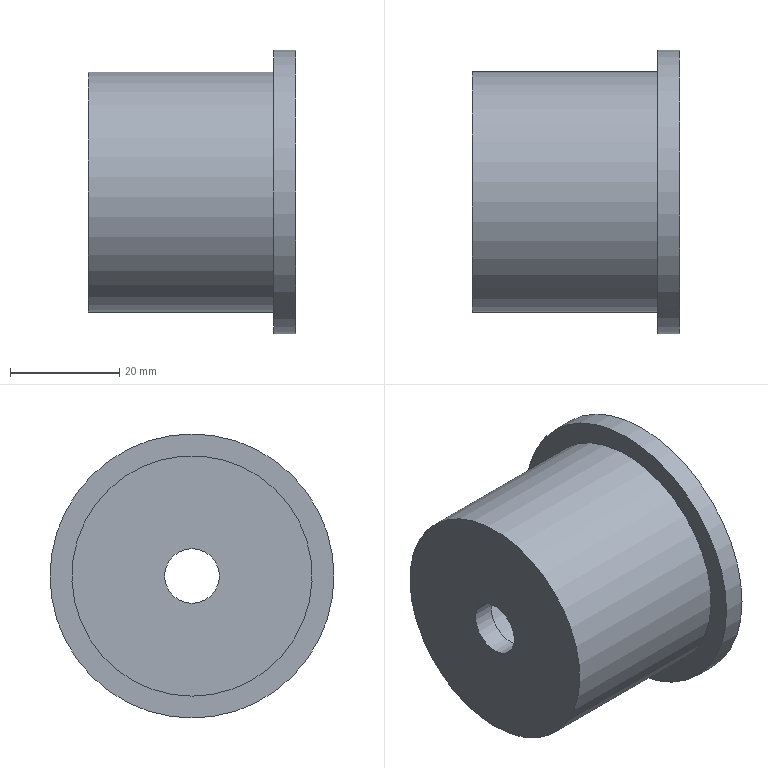Component | NX | LARGE_SPRING_BASE_2 | 1 solid | 10 faces | box 38 x 52 x 52 mm | volume 38909 mm3 | plane 5 | cylinder 5 | commonest cylinder face diameters 10 x1 26 x1 36 x1 52 x1 44 x1
STEP:
#1=CARTESIAN_POINT('',(0.,0.,0.));
#2=DIRECTION('',(0.,0.,1.));
#3=DIRECTION('',(1.,0.,0.));
#4=AXIS2_PLACEMENT_3D('',#1,#2,#3);
#5=CARTESIAN_POINT('',(-43.003,0.,-5.));
#6=VERTEX_POINT('',#5);
#7=CARTESIAN_POINT('',(-43.003,0.,0.));
#8=DIRECTION('',(-1.,0.,0.));
#9=DIRECTION('',(0.,0.,-1.));
#10=AXIS2_PLACEMENT_3D('',#7,#8,#9);
#11=CIRCLE('',#10,5.);
#12=CARTESIAN_POINT('',(-43.003,0.,22.));
#13=DIRECTION('',(1.,0.,0.));
#14=DIRECTION('',(0.,0.,1.));
#15=AXIS2_PLACEMENT_3D('',#12,#13,#14);
#16=PLANE('',#15);
#17=CARTESIAN_POINT('',(-27.,0.));
#18=CARTESIAN_POINT('',(-27.,8.66));
#19=CARTESIAN_POINT('',(-19.5,4.33));
#20=CARTESIAN_POINT('',(-12.,0.));
#21=CARTESIAN_POINT('',(-19.5,-4.33));
#22=CARTESIAN_POINT('',(-27.,-8.66));
#23=CARTESIAN_POINT('',(-27.,0.));
#24=(BOUNDED_CURVE()B_SPLINE_CURVE(2,(#17,#18,#19,#20,#21,#22,#23),.UNSPECIFIED.,.T.,.F.)B_SPLINE_CURVE_WITH_KNOTS((1,2,2,2,2,1),(-2.094,0.,2.094,4.189,6.283,8.378),.UNSPECIFIED.)CURVE()GEOMETRIC_REPRESENTATION_ITEM()RATIONAL_B_SPLINE_CURVE((1.,0.5,1.,0.5,1.,0.5,1.))REPRESENTATION_ITEM(''));
#25=(GEOMETRIC_REPRESENTATION_CONTEXT(2)PARAMETRIC_REPRESENTATION_CONTEXT()REPRESENTATION_CONTEXT('',''));
#26=DEFINITIONAL_REPRESENTATION('',(#24),#25);
#27=PCURVE('',#16,#26);
#28=CARTESIAN_POINT('',(-5.,0.,0.));
#29=DIRECTION('',(-1.,0.,0.));
#30=DIRECTION('',(0.,0.,-1.));
#31=AXIS2_PLACEMENT_3D('',#28,#29,#30);
#32=CYLINDRICAL_SURFACE('',#31,5.);
#33=CARTESIAN_POINT('',(0.,38.003));
#34=DIRECTION('',(1.,0.));
#35=VECTOR('',#34,1.);
#36=LINE('',#33,#35);
#37=(GEOMETRIC_REPRESENTATION_CONTEXT(2)PARAMETRIC_REPRESENTATION_CONTEXT()REPRESENTATION_CONTEXT('',''));
#38=DEFINITIONAL_REPRESENTATION('',(#36),#37);
#39=PCURVE('',#32,#38);
#40=SURFACE_CURVE('',#11,(#27,#39),.PCURVE_S1.);
#41=EDGE_CURVE('',#6,#6,#40,.T.);
#42=ORIENTED_EDGE('',*,*,#41,.F.);
#43=EDGE_LOOP('',(#42));
#44=FACE_BOUND('',#43,.T.);
#45=CARTESIAN_POINT('',(-43.003,0.,-22.));
#46=VERTEX_POINT('',#45);
#47=CARTESIAN_POINT('',(-43.003,0.,0.));
#48=DIRECTION('',(-1.,0.,0.));
#49=DIRECTION('',(0.,0.,-1.));
#50=AXIS2_PLACEMENT_3D('',#47,#48,#49);
#51=CIRCLE('',#50,22.);
#52=CARTESIAN_POINT('',(-44.,0.));
#53=CARTESIAN_POINT('',(-44.,38.105));
#54=CARTESIAN_POINT('',(-11.,19.053));
#55=CARTESIAN_POINT('',(22.,0.));
#56=CARTESIAN_POINT('',(-11.,-19.053));
#57=CARTESIAN_POINT('',(-44.,-38.105));
#58=CARTESIAN_POINT('',(-44.,0.));
#59=(BOUNDED_CURVE()B_SPLINE_CURVE(2,(#52,#53,#54,#55,#56,#57,#58),.UNSPECIFIED.,.T.,.F.)B_SPLINE_CURVE_WITH_KNOTS((1,2,2,2,2,1),(-2.094,0.,2.094,4.189,6.283,8.378),.UNSPECIFIED.)CURVE()GEOMETRIC_REPRESENTATION_ITEM()RATIONAL_B_SPLINE_CURVE((1.,0.5,1.,0.5,1.,0.5,1.))REPRESENTATION_ITEM(''));
#60=(GEOMETRIC_REPRESENTATION_CONTEXT(2)PARAMETRIC_REPRESENTATION_CONTEXT()REPRESENTATION_CONTEXT('',''));
#61=DEFINITIONAL_REPRESENTATION('',(#59),#60);
#62=PCURVE('',#16,#61);
#63=CARTESIAN_POINT('',(-5.,0.,0.));
#64=DIRECTION('',(-1.,0.,0.));
#65=DIRECTION('',(0.,0.,-1.));
#66=AXIS2_PLACEMENT_3D('',#63,#64,#65);
#67=CYLINDRICAL_SURFACE('',#66,22.);
#68=CARTESIAN_POINT('',(0.,38.003));
#69=DIRECTION('',(1.,0.));
#70=VECTOR('',#69,1.);
#71=LINE('',#68,#70);
#72=(GEOMETRIC_REPRESENTATION_CONTEXT(2)PARAMETRIC_REPRESENTATION_CONTEXT()REPRESENTATION_CONTEXT('',''));
#73=DEFINITIONAL_REPRESENTATION('',(#71),#72);
#74=PCURVE('',#67,#73);
#75=SURFACE_CURVE('',#51,(#62,#74),.PCURVE_S1.);
#76=EDGE_CURVE('',#46,#46,#75,.T.);
#77=ORIENTED_EDGE('',*,*,#76,.T.);
#78=EDGE_LOOP('',(#77));
#79=FACE_BOUND('',#78,.T.);
#80=ADVANCED_FACE('',(#44,#79),#16,.F.);
#81=CARTESIAN_POINT('',(-39.003,0.,-5.));
#82=VERTEX_POINT('',#81);
#83=CARTESIAN_POINT('',(-39.003,0.,0.));
#84=DIRECTION('',(-1.,0.,0.));
#85=DIRECTION('',(0.,0.,-1.));
#86=AXIS2_PLACEMENT_3D('',#83,#84,#85);
#87=CIRCLE('',#86,5.);
#88=CARTESIAN_POINT('',(0.,34.003));
#89=DIRECTION('',(1.,0.));
#90=VECTOR('',#89,1.);
#91=LINE('',#88,#90);
#92=(GEOMETRIC_REPRESENTATION_CONTEXT(2)PARAMETRIC_REPRESENTATION_CONTEXT()REPRESENTATION_CONTEXT('',''));
#93=DEFINITIONAL_REPRESENTATION('',(#91),#92);
#94=PCURVE('',#32,#93);
#95=CARTESIAN_POINT('',(-39.003,0.,5.));
#96=DIRECTION('',(-1.,0.,0.));
#97=DIRECTION('',(0.,0.,-1.));
#98=AXIS2_PLACEMENT_3D('',#95,#96,#97);
#99=PLANE('',#98);
#100=CARTESIAN_POINT('',(5.,0.));
#101=DIRECTION('',(1.,0.));
#102=AXIS2_PLACEMENT_2D('',#100,#101);
#103=CIRCLE('',#102,5.);
#104=(GEOMETRIC_REPRESENTATION_CONTEXT(2)PARAMETRIC_REPRESENTATION_CONTEXT()REPRESENTATION_CONTEXT('',''));
#105=DEFINITIONAL_REPRESENTATION('',(#103),#104);
#106=PCURVE('',#99,#105);
#107=SURFACE_CURVE('',#87,(#94,#106),.PCURVE_S1.);
#108=EDGE_CURVE('',#82,#82,#107,.T.);
#109=ORIENTED_EDGE('',*,*,#108,.T.);
#110=CARTESIAN_POINT('',(-39.003,0.,-5.));
#111=CARTESIAN_POINT('',(-43.003,0.,-5.));
#112=B_SPLINE_CURVE_WITH_KNOTS('',1,(#110,#111),.UNSPECIFIED.,.F.,.F.,(2,2),(34.003,38.003),.PIECEWISE_BEZIER_KNOTS.);
#113=CARTESIAN_POINT('',(6.283,0.));
#114=DIRECTION('',(0.,1.));
#115=VECTOR('',#114,1.);
#116=LINE('',#113,#115);
#117=(GEOMETRIC_REPRESENTATION_CONTEXT(2)PARAMETRIC_REPRESENTATION_CONTEXT()REPRESENTATION_CONTEXT('',''));
#118=DEFINITIONAL_REPRESENTATION('',(#116),#117);
#119=PCURVE('',#32,#118);
#120=CARTESIAN_POINT('',(0.,0.));
#121=DIRECTION('',(0.,1.));
#122=VECTOR('',#121,1.);
#123=LINE('',#120,#122);
#124=(GEOMETRIC_REPRESENTATION_CONTEXT(2)PARAMETRIC_REPRESENTATION_CONTEXT()REPRESENTATION_CONTEXT('',''));
#125=DEFINITIONAL_REPRESENTATION('',(#123),#124);
#126=PCURVE('',#32,#125);
#127=SEAM_CURVE('',#112,(#119,#126),.PCURVE_S1.);
#128=EDGE_CURVE('',#82,#6,#127,.T.);
#129=ORIENTED_EDGE('',*,*,#128,.T.);
#130=ORIENTED_EDGE('',*,*,#41,.F.);
#131=ORIENTED_EDGE('',*,*,#128,.F.);
#132=EDGE_LOOP('',(#109,#129,#130,#131));
#133=FACE_BOUND('',#132,.F.);
#134=ADVANCED_FACE('',(#133),#32,.F.);
#135=CARTESIAN_POINT('',(-39.003,0.,-13.));
#136=VERTEX_POINT('',#135);
#137=CARTESIAN_POINT('',(-39.003,0.,0.));
#138=DIRECTION('',(-1.,0.,0.));
#139=DIRECTION('',(0.,0.,-1.));
#140=AXIS2_PLACEMENT_3D('',#137,#138,#139);
#141=CIRCLE('',#140,13.);
#142=CARTESIAN_POINT('',(5.,0.));
#143=DIRECTION('',(1.,0.));
#144=AXIS2_PLACEMENT_2D('',#142,#143);
#145=CIRCLE('',#144,13.);
#146=(GEOMETRIC_REPRESENTATION_CONTEXT(2)PARAMETRIC_REPRESENTATION_CONTEXT()REPRESENTATION_CONTEXT('',''));
#147=DEFINITIONAL_REPRESENTATION('',(#145),#146);
#148=PCURVE('',#99,#147);
#149=CARTESIAN_POINT('',(-5.,0.,0.));
#150=DIRECTION('',(-1.,0.,0.));
#151=DIRECTION('',(0.,0.,-1.));
#152=AXIS2_PLACEMENT_3D('',#149,#150,#151);
#153=CYLINDRICAL_SURFACE('',#152,13.);
#154=CARTESIAN_POINT('',(0.,34.003));
#155=DIRECTION('',(1.,0.));
#156=VECTOR('',#155,1.);
#157=LINE('',#154,#156);
#158=(GEOMETRIC_REPRESENTATION_CONTEXT(2)PARAMETRIC_REPRESENTATION_CONTEXT()REPRESENTATION_CONTEXT('',''));
#159=DEFINITIONAL_REPRESENTATION('',(#157),#158);
#160=PCURVE('',#153,#159);
#161=SURFACE_CURVE('',#141,(#148,#160),.PCURVE_S1.);
#162=EDGE_CURVE('',#136,#136,#161,.T.);
#163=ORIENTED_EDGE('',*,*,#162,.F.);
#164=EDGE_LOOP('',(#163));
#165=FACE_BOUND('',#164,.T.);
#166=ORIENTED_EDGE('',*,*,#108,.T.);
#167=EDGE_LOOP('',(#166));
#168=FACE_BOUND('',#167,.T.);
#169=ADVANCED_FACE('',(#165,#168),#99,.F.);
#170=CARTESIAN_POINT('',(-11.003,0.,-13.));
#171=VERTEX_POINT('',#170);
#172=CARTESIAN_POINT('',(-11.003,0.,0.));
#173=DIRECTION('',(-1.,0.,0.));
#174=DIRECTION('',(0.,0.,-1.));
#175=AXIS2_PLACEMENT_3D('',#172,#173,#174);
#176=CIRCLE('',#175,13.);
#177=CARTESIAN_POINT('',(0.,6.003));
#178=DIRECTION('',(1.,0.));
#179=VECTOR('',#178,1.);
#180=LINE('',#177,#179);
#181=(GEOMETRIC_REPRESENTATION_CONTEXT(2)PARAMETRIC_REPRESENTATION_CONTEXT()REPRESENTATION_CONTEXT('',''));
#182=DEFINITIONAL_REPRESENTATION('',(#180),#181);
#183=PCURVE('',#153,#182);
#184=CARTESIAN_POINT('',(-11.003,0.,13.));
#185=DIRECTION('',(-1.,0.,0.));
#186=DIRECTION('',(0.,0.,-1.));
#187=AXIS2_PLACEMENT_3D('',#184,#185,#186);
#188=PLANE('',#187);
#189=CARTESIAN_POINT('',(13.,0.));
#190=DIRECTION('',(1.,0.));
#191=AXIS2_PLACEMENT_2D('',#189,#190);
#192=CIRCLE('',#191,13.);
#193=(GEOMETRIC_REPRESENTATION_CONTEXT(2)PARAMETRIC_REPRESENTATION_CONTEXT()REPRESENTATION_CONTEXT('',''));
#194=DEFINITIONAL_REPRESENTATION('',(#192),#193);
#195=PCURVE('',#188,#194);
#196=SURFACE_CURVE('',#176,(#183,#195),.PCURVE_S1.);
#197=EDGE_CURVE('',#171,#171,#196,.T.);
#198=ORIENTED_EDGE('',*,*,#197,.T.);
#199=CARTESIAN_POINT('',(-11.003,0.,-13.));
#200=CARTESIAN_POINT('',(-39.003,0.,-13.));
#201=B_SPLINE_CURVE_WITH_KNOTS('',1,(#199,#200),.UNSPECIFIED.,.F.,.F.,(2,2),(6.003,34.003),.PIECEWISE_BEZIER_KNOTS.);
#202=CARTESIAN_POINT('',(6.283,0.));
#203=DIRECTION('',(0.,1.));
#204=VECTOR('',#203,1.);
#205=LINE('',#202,#204);
#206=(GEOMETRIC_REPRESENTATION_CONTEXT(2)PARAMETRIC_REPRESENTATION_CONTEXT()REPRESENTATION_CONTEXT('',''));
#207=DEFINITIONAL_REPRESENTATION('',(#205),#206);
#208=PCURVE('',#153,#207);
#209=CARTESIAN_POINT('',(0.,0.));
#210=DIRECTION('',(0.,1.));
#211=VECTOR('',#210,1.);
#212=LINE('',#209,#211);
#213=(GEOMETRIC_REPRESENTATION_CONTEXT(2)PARAMETRIC_REPRESENTATION_CONTEXT()REPRESENTATION_CONTEXT('',''));
#214=DEFINITIONAL_REPRESENTATION('',(#212),#213);
#215=PCURVE('',#153,#214);
#216=SEAM_CURVE('',#201,(#208,#215),.PCURVE_S1.);
#217=EDGE_CURVE('',#171,#136,#216,.T.);
#218=ORIENTED_EDGE('',*,*,#217,.T.);
#219=ORIENTED_EDGE('',*,*,#162,.F.);
#220=ORIENTED_EDGE('',*,*,#217,.F.);
#221=EDGE_LOOP('',(#198,#218,#219,#220));
#222=FACE_BOUND('',#221,.F.);
#223=ADVANCED_FACE('',(#222),#153,.F.);
#224=CARTESIAN_POINT('',(-11.003,0.,-18.));
#225=VERTEX_POINT('',#224);
#226=CARTESIAN_POINT('',(-11.003,0.,0.));
#227=DIRECTION('',(-1.,0.,0.));
#228=DIRECTION('',(0.,0.,-1.));
#229=AXIS2_PLACEMENT_3D('',#226,#227,#228);
#230=CIRCLE('',#229,18.);
#231=CARTESIAN_POINT('',(13.,0.));
#232=DIRECTION('',(1.,0.));
#233=AXIS2_PLACEMENT_2D('',#231,#232);
#234=CIRCLE('',#233,18.);
#235=(GEOMETRIC_REPRESENTATION_CONTEXT(2)PARAMETRIC_REPRESENTATION_CONTEXT()REPRESENTATION_CONTEXT('',''));
#236=DEFINITIONAL_REPRESENTATION('',(#234),#235);
#237=PCURVE('',#188,#236);
#238=CARTESIAN_POINT('',(-5.,0.,0.));
#239=DIRECTION('',(-1.,0.,0.));
#240=DIRECTION('',(0.,0.,-1.));
#241=AXIS2_PLACEMENT_3D('',#238,#239,#240);
#242=CYLINDRICAL_SURFACE('',#241,18.);
#243=CARTESIAN_POINT('',(0.,6.003));
#244=DIRECTION('',(1.,0.));
#245=VECTOR('',#244,1.);
#246=LINE('',#243,#245);
#247=(GEOMETRIC_REPRESENTATION_CONTEXT(2)PARAMETRIC_REPRESENTATION_CONTEXT()REPRESENTATION_CONTEXT('',''));
#248=DEFINITIONAL_REPRESENTATION('',(#246),#247);
#249=PCURVE('',#242,#248);
#250=SURFACE_CURVE('',#230,(#237,#249),.PCURVE_S1.);
#251=EDGE_CURVE('',#225,#225,#250,.T.);
#252=ORIENTED_EDGE('',*,*,#251,.F.);
#253=EDGE_LOOP('',(#252));
#254=FACE_BOUND('',#253,.T.);
#255=ORIENTED_EDGE('',*,*,#197,.T.);
#256=EDGE_LOOP('',(#255));
#257=FACE_BOUND('',#256,.T.);
#258=ADVANCED_FACE('',(#254,#257),#188,.F.);
#259=CARTESIAN_POINT('',(-5.,0.,-18.));
#260=VERTEX_POINT('',#259);
#261=CARTESIAN_POINT('',(-5.,0.,0.));
#262=DIRECTION('',(-1.,0.,0.));
#263=DIRECTION('',(0.,0.,-1.));
#264=AXIS2_PLACEMENT_3D('',#261,#262,#263);
#265=CIRCLE('',#264,18.);
#266=CARTESIAN_POINT('',(0.,0.));
#267=DIRECTION('',(1.,0.));
#268=VECTOR('',#267,1.);
#269=LINE('',#266,#268);
#270=(GEOMETRIC_REPRESENTATION_CONTEXT(2)PARAMETRIC_REPRESENTATION_CONTEXT()REPRESENTATION_CONTEXT('',''));
#271=DEFINITIONAL_REPRESENTATION('',(#269),#270);
#272=PCURVE('',#242,#271);
#273=CARTESIAN_POINT('',(-5.,0.,18.));
#274=DIRECTION('',(-1.,0.,0.));
#275=DIRECTION('',(0.,0.,-1.));
#276=AXIS2_PLACEMENT_3D('',#273,#274,#275);
#277=PLANE('',#276);
#278=CARTESIAN_POINT('',(18.,0.));
#279=DIRECTION('',(1.,0.));
#280=AXIS2_PLACEMENT_2D('',#278,#279);
#281=CIRCLE('',#280,18.);
#282=(GEOMETRIC_REPRESENTATION_CONTEXT(2)PARAMETRIC_REPRESENTATION_CONTEXT()REPRESENTATION_CONTEXT('',''));
#283=DEFINITIONAL_REPRESENTATION('',(#281),#282);
#284=PCURVE('',#277,#283);
#285=SURFACE_CURVE('',#265,(#272,#284),.PCURVE_S1.);
#286=EDGE_CURVE('',#260,#260,#285,.T.);
#287=ORIENTED_EDGE('',*,*,#286,.T.);
#288=CARTESIAN_POINT('',(-5.,0.,-18.));
#289=CARTESIAN_POINT('',(-11.003,0.,-18.));
#290=B_SPLINE_CURVE_WITH_KNOTS('',1,(#288,#289),.UNSPECIFIED.,.F.,.F.,(2,2),(0.,6.003),.PIECEWISE_BEZIER_KNOTS.);
#291=CARTESIAN_POINT('',(6.283,0.));
#292=DIRECTION('',(0.,1.));
#293=VECTOR('',#292,1.);
#294=LINE('',#291,#293);
#295=(GEOMETRIC_REPRESENTATION_CONTEXT(2)PARAMETRIC_REPRESENTATION_CONTEXT()REPRESENTATION_CONTEXT('',''));
#296=DEFINITIONAL_REPRESENTATION('',(#294),#295);
#297=PCURVE('',#242,#296);
#298=CARTESIAN_POINT('',(0.,0.));
#299=DIRECTION('',(0.,1.));
#300=VECTOR('',#299,1.);
#301=LINE('',#298,#300);
#302=(GEOMETRIC_REPRESENTATION_CONTEXT(2)PARAMETRIC_REPRESENTATION_CONTEXT()REPRESENTATION_CONTEXT('',''));
#303=DEFINITIONAL_REPRESENTATION('',(#301),#302);
#304=PCURVE('',#242,#303);
#305=SEAM_CURVE('',#290,(#297,#304),.PCURVE_S1.);
#306=EDGE_CURVE('',#260,#225,#305,.T.);
#307=ORIENTED_EDGE('',*,*,#306,.T.);
#308=ORIENTED_EDGE('',*,*,#251,.F.);
#309=ORIENTED_EDGE('',*,*,#306,.F.);
#310=EDGE_LOOP('',(#287,#307,#308,#309));
#311=FACE_BOUND('',#310,.F.);
#312=ADVANCED_FACE('',(#311),#242,.F.);
#313=CARTESIAN_POINT('',(-5.,0.,-26.));
#314=VERTEX_POINT('',#313);
#315=CARTESIAN_POINT('',(-5.,0.,0.));
#316=DIRECTION('',(-1.,0.,0.));
#317=DIRECTION('',(0.,0.,-1.));
#318=AXIS2_PLACEMENT_3D('',#315,#316,#317);
#319=CIRCLE('',#318,26.);
#320=CARTESIAN_POINT('',(18.,0.));
#321=DIRECTION('',(1.,0.));
#322=AXIS2_PLACEMENT_2D('',#320,#321);
#323=CIRCLE('',#322,26.);
#324=(GEOMETRIC_REPRESENTATION_CONTEXT(2)PARAMETRIC_REPRESENTATION_CONTEXT()REPRESENTATION_CONTEXT('',''));
#325=DEFINITIONAL_REPRESENTATION('',(#323),#324);
#326=PCURVE('',#277,#325);
#327=CARTESIAN_POINT('',(-5.,0.,0.));
#328=DIRECTION('',(-1.,0.,0.));
#329=DIRECTION('',(0.,0.,-1.));
#330=AXIS2_PLACEMENT_3D('',#327,#328,#329);
#331=CYLINDRICAL_SURFACE('',#330,26.);
#332=CARTESIAN_POINT('',(0.,0.));
#333=DIRECTION('',(1.,0.));
#334=VECTOR('',#333,1.);
#335=LINE('',#332,#334);
#336=(GEOMETRIC_REPRESENTATION_CONTEXT(2)PARAMETRIC_REPRESENTATION_CONTEXT()REPRESENTATION_CONTEXT('',''));
#337=DEFINITIONAL_REPRESENTATION('',(#335),#336);
#338=PCURVE('',#331,#337);
#339=SURFACE_CURVE('',#319,(#326,#338),.PCURVE_S1.);
#340=EDGE_CURVE('',#314,#314,#339,.T.);
#341=ORIENTED_EDGE('',*,*,#340,.F.);
#342=EDGE_LOOP('',(#341));
#343=FACE_BOUND('',#342,.T.);
#344=ORIENTED_EDGE('',*,*,#286,.T.);
#345=EDGE_LOOP('',(#344));
#346=FACE_BOUND('',#345,.T.);
#347=ADVANCED_FACE('',(#343,#346),#277,.F.);
#348=CARTESIAN_POINT('',(-9.003,0.,-26.));
#349=VERTEX_POINT('',#348);
#350=CARTESIAN_POINT('',(-9.003,0.,0.));
#351=DIRECTION('',(-1.,0.,0.));
#352=DIRECTION('',(0.,0.,-1.));
#353=AXIS2_PLACEMENT_3D('',#350,#351,#352);
#354=CIRCLE('',#353,26.);
#355=CARTESIAN_POINT('',(0.,4.003));
#356=DIRECTION('',(1.,0.));
#357=VECTOR('',#356,1.);
#358=LINE('',#355,#357);
#359=(GEOMETRIC_REPRESENTATION_CONTEXT(2)PARAMETRIC_REPRESENTATION_CONTEXT()REPRESENTATION_CONTEXT('',''));
#360=DEFINITIONAL_REPRESENTATION('',(#358),#359);
#361=PCURVE('',#331,#360);
#362=CARTESIAN_POINT('',(-9.003,0.,26.));
#363=DIRECTION('',(1.,0.,0.));
#364=DIRECTION('',(0.,0.,1.));
#365=AXIS2_PLACEMENT_3D('',#362,#363,#364);
#366=PLANE('',#365);
#367=CARTESIAN_POINT('',(-52.,0.));
#368=CARTESIAN_POINT('',(-52.,45.033));
#369=CARTESIAN_POINT('',(-13.,22.517));
#370=CARTESIAN_POINT('',(26.,0.));
#371=CARTESIAN_POINT('',(-13.,-22.517));
#372=CARTESIAN_POINT('',(-52.,-45.033));
#373=CARTESIAN_POINT('',(-52.,0.));
#374=(BOUNDED_CURVE()B_SPLINE_CURVE(2,(#367,#368,#369,#370,#371,#372,#373),.UNSPECIFIED.,.T.,.F.)B_SPLINE_CURVE_WITH_KNOTS((1,2,2,2,2,1),(-2.094,0.,2.094,4.189,6.283,8.378),.UNSPECIFIED.)CURVE()GEOMETRIC_REPRESENTATION_ITEM()RATIONAL_B_SPLINE_CURVE((1.,0.5,1.,0.5,1.,0.5,1.))REPRESENTATION_ITEM(''));
#375=(GEOMETRIC_REPRESENTATION_CONTEXT(2)PARAMETRIC_REPRESENTATION_CONTEXT()REPRESENTATION_CONTEXT('',''));
#376=DEFINITIONAL_REPRESENTATION('',(#374),#375);
#377=PCURVE('',#366,#376);
#378=SURFACE_CURVE('',#354,(#361,#377),.PCURVE_S1.);
#379=EDGE_CURVE('',#349,#349,#378,.T.);
#380=ORIENTED_EDGE('',*,*,#379,.F.);
#381=CARTESIAN_POINT('',(-5.,0.,-26.));
#382=CARTESIAN_POINT('',(-9.003,0.,-26.));
#383=B_SPLINE_CURVE_WITH_KNOTS('',1,(#381,#382),.UNSPECIFIED.,.F.,.F.,(2,2),(0.,4.003),.PIECEWISE_BEZIER_KNOTS.);
#384=CARTESIAN_POINT('',(0.,0.));
#385=DIRECTION('',(0.,1.));
#386=VECTOR('',#385,1.);
#387=LINE('',#384,#386);
#388=(GEOMETRIC_REPRESENTATION_CONTEXT(2)PARAMETRIC_REPRESENTATION_CONTEXT()REPRESENTATION_CONTEXT('',''));
#389=DEFINITIONAL_REPRESENTATION('',(#387),#388);
#390=PCURVE('',#331,#389);
#391=CARTESIAN_POINT('',(6.283,0.));
#392=DIRECTION('',(0.,1.));
#393=VECTOR('',#392,1.);
#394=LINE('',#391,#393);
#395=(GEOMETRIC_REPRESENTATION_CONTEXT(2)PARAMETRIC_REPRESENTATION_CONTEXT()REPRESENTATION_CONTEXT('',''));
#396=DEFINITIONAL_REPRESENTATION('',(#394),#395);
#397=PCURVE('',#331,#396);
#398=SEAM_CURVE('',#383,(#390,#397),.PCURVE_S1.);
#399=EDGE_CURVE('',#314,#349,#398,.T.);
#400=ORIENTED_EDGE('',*,*,#399,.F.);
#401=ORIENTED_EDGE('',*,*,#340,.T.);
#402=ORIENTED_EDGE('',*,*,#399,.T.);
#403=EDGE_LOOP('',(#380,#400,#401,#402));
#404=FACE_BOUND('',#403,.T.);
#405=ADVANCED_FACE('',(#404),#331,.T.);
#406=CARTESIAN_POINT('',(-9.003,0.,-22.));
#407=VERTEX_POINT('',#406);
#408=CARTESIAN_POINT('',(-9.003,0.,0.));
#409=DIRECTION('',(-1.,0.,0.));
#410=DIRECTION('',(0.,0.,-1.));
#411=AXIS2_PLACEMENT_3D('',#408,#409,#410);
#412=CIRCLE('',#411,22.);
#413=CARTESIAN_POINT('',(-48.,0.));
#414=CARTESIAN_POINT('',(-48.,38.105));
#415=CARTESIAN_POINT('',(-15.,19.053));
#416=CARTESIAN_POINT('',(18.,0.));
#417=CARTESIAN_POINT('',(-15.,-19.053));
#418=CARTESIAN_POINT('',(-48.,-38.105));
#419=CARTESIAN_POINT('',(-48.,0.));
#420=(BOUNDED_CURVE()B_SPLINE_CURVE(2,(#413,#414,#415,#416,#417,#418,#419),.UNSPECIFIED.,.T.,.F.)B_SPLINE_CURVE_WITH_KNOTS((1,2,2,2,2,1),(-2.094,0.,2.094,4.189,6.283,8.378),.UNSPECIFIED.)CURVE()GEOMETRIC_REPRESENTATION_ITEM()RATIONAL_B_SPLINE_CURVE((1.,0.5,1.,0.5,1.,0.5,1.))REPRESENTATION_ITEM(''));
#421=(GEOMETRIC_REPRESENTATION_CONTEXT(2)PARAMETRIC_REPRESENTATION_CONTEXT()REPRESENTATION_CONTEXT('',''));
#422=DEFINITIONAL_REPRESENTATION('',(#420),#421);
#423=PCURVE('',#366,#422);
#424=CARTESIAN_POINT('',(0.,4.003));
#425=DIRECTION('',(1.,0.));
#426=VECTOR('',#425,1.);
#427=LINE('',#424,#426);
#428=(GEOMETRIC_REPRESENTATION_CONTEXT(2)PARAMETRIC_REPRESENTATION_CONTEXT()REPRESENTATION_CONTEXT('',''));
#429=DEFINITIONAL_REPRESENTATION('',(#427),#428);
#430=PCURVE('',#67,#429);
#431=SURFACE_CURVE('',#412,(#423,#430),.PCURVE_S1.);
#432=EDGE_CURVE('',#407,#407,#431,.T.);
#433=ORIENTED_EDGE('',*,*,#432,.F.);
#434=EDGE_LOOP('',(#433));
#435=FACE_BOUND('',#434,.T.);
#436=ORIENTED_EDGE('',*,*,#379,.T.);
#437=EDGE_LOOP('',(#436));
#438=FACE_BOUND('',#437,.T.);
#439=ADVANCED_FACE('',(#435,#438),#366,.F.);
#440=ORIENTED_EDGE('',*,*,#76,.F.);
#441=CARTESIAN_POINT('',(-9.003,0.,-22.));
#442=CARTESIAN_POINT('',(-43.003,0.,-22.));
#443=B_SPLINE_CURVE_WITH_KNOTS('',1,(#441,#442),.UNSPECIFIED.,.F.,.F.,(2,2),(4.003,38.003),.PIECEWISE_BEZIER_KNOTS.);
#444=CARTESIAN_POINT('',(0.,0.));
#445=DIRECTION('',(0.,1.));
#446=VECTOR('',#445,1.);
#447=LINE('',#444,#446);
#448=(GEOMETRIC_REPRESENTATION_CONTEXT(2)PARAMETRIC_REPRESENTATION_CONTEXT()REPRESENTATION_CONTEXT('',''));
#449=DEFINITIONAL_REPRESENTATION('',(#447),#448);
#450=PCURVE('',#67,#449);
#451=CARTESIAN_POINT('',(6.283,0.));
#452=DIRECTION('',(0.,1.));
#453=VECTOR('',#452,1.);
#454=LINE('',#451,#453);
#455=(GEOMETRIC_REPRESENTATION_CONTEXT(2)PARAMETRIC_REPRESENTATION_CONTEXT()REPRESENTATION_CONTEXT('',''));
#456=DEFINITIONAL_REPRESENTATION('',(#454),#455);
#457=PCURVE('',#67,#456);
#458=SEAM_CURVE('',#443,(#450,#457),.PCURVE_S1.);
#459=EDGE_CURVE('',#407,#46,#458,.T.);
#460=ORIENTED_EDGE('',*,*,#459,.F.);
#461=ORIENTED_EDGE('',*,*,#432,.T.);
#462=ORIENTED_EDGE('',*,*,#459,.T.);
#463=EDGE_LOOP('',(#440,#460,#461,#462));
#464=FACE_BOUND('',#463,.T.);
#465=ADVANCED_FACE('',(#464),#67,.T.);
#466=CLOSED_SHELL('',(#80,#134,#169,#223,#258,#312,#347,#405,#439,#465));
#467=MANIFOLD_SOLID_BREP('',#466);
#468=(LENGTH_UNIT()NAMED_UNIT(*)SI_UNIT(.MILLI.,.METRE.));
#469=UNCERTAINTY_MEASURE_WITH_UNIT(LENGTH_MEASURE(0.00001),#468,'','');
#470=(NAMED_UNIT(*)PLANE_ANGLE_UNIT()SI_UNIT($,.RADIAN.));
#471=(NAMED_UNIT(*)SI_UNIT($,.STERADIAN.)SOLID_ANGLE_UNIT());
#472=(GEOMETRIC_REPRESENTATION_CONTEXT(3)GLOBAL_UNCERTAINTY_ASSIGNED_CONTEXT((#469))GLOBAL_UNIT_ASSIGNED_CONTEXT((#468,#470,#471))REPRESENTATION_CONTEXT('',''));
#473=ADVANCED_BREP_SHAPE_REPRESENTATION('',(#4,#467),#472);